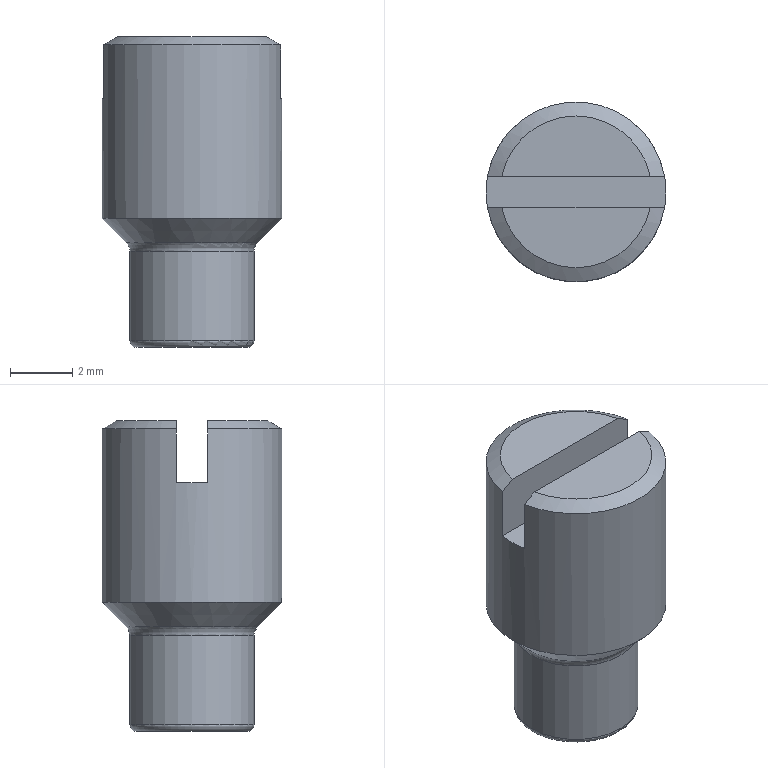Component | NX | SET_SCREW | 1 solid | 13 faces | box 5.8 x 5.8 x 10 mm | volume 200 mm3 | plane 6 | cone 3 | cylinder 2 | torus 2 | commonest cylinder face diameters 5.795 x1 4 x1
STEP:
#1=CARTESIAN_POINT('',(0.,0.,0.));
#2=DIRECTION('',(0.,0.,1.));
#3=DIRECTION('',(1.,0.,0.));
#4=AXIS2_PLACEMENT_3D('',#1,#2,#3);
#5=CARTESIAN_POINT('',(55.394,0.5,23.5));
#6=VERTEX_POINT('',#5);
#7=CARTESIAN_POINT('',(50.606,0.5,23.5));
#8=VERTEX_POINT('',#7);
#9=CARTESIAN_POINT('',(58.795,0.5,23.5));
#10=DIRECTION('',(-1.,0.,0.));
#11=VECTOR('',#10,1.);
#12=LINE('',#9,#11);
#13=CARTESIAN_POINT('',(53.,2.446,23.5));
#14=DIRECTION('',(0.,0.,-1.));
#15=DIRECTION('',(-1.,0.,0.));
#16=AXIS2_PLACEMENT_3D('',#13,#14,#15);
#17=PLANE('',#16);
#18=CARTESIAN_POINT('',(-5.795,-1.946));
#19=DIRECTION('',(1.,0.));
#20=VECTOR('',#19,1.);
#21=LINE('',#18,#20);
#22=(GEOMETRIC_REPRESENTATION_CONTEXT(2)PARAMETRIC_REPRESENTATION_CONTEXT()REPRESENTATION_CONTEXT('',''));
#23=DEFINITIONAL_REPRESENTATION('',(#21),#22);
#24=PCURVE('',#17,#23);
#25=CARTESIAN_POINT('',(58.795,0.5,23.5));
#26=DIRECTION('',(0.,1.,0.));
#27=DIRECTION('',(0.,-0.,1.));
#28=AXIS2_PLACEMENT_3D('',#25,#26,#27);
#29=PLANE('',#28);
#30=CARTESIAN_POINT('',(0.,0.));
#31=DIRECTION('',(0.,-1.));
#32=VECTOR('',#31,1.);
#33=LINE('',#30,#32);
#34=(GEOMETRIC_REPRESENTATION_CONTEXT(2)PARAMETRIC_REPRESENTATION_CONTEXT()REPRESENTATION_CONTEXT('',''));
#35=DEFINITIONAL_REPRESENTATION('',(#33),#34);
#36=PCURVE('',#29,#35);
#37=SURFACE_CURVE('',#12,(#24,#36),.PCURVE_S1.);
#38=EDGE_CURVE('',#6,#8,#37,.T.);
#39=ORIENTED_EDGE('',*,*,#38,.F.);
#40=CARTESIAN_POINT('',(53.,-0.,23.5));
#41=DIRECTION('',(0.,0.,1.));
#42=DIRECTION('',(1.,0.,0.));
#43=AXIS2_PLACEMENT_3D('',#40,#41,#42);
#44=CIRCLE('',#43,2.446);
#45=CARTESIAN_POINT('',(-2.446,-2.446));
#46=CARTESIAN_POINT('',(-2.446,1.79));
#47=CARTESIAN_POINT('',(1.223,-0.3276));
#48=CARTESIAN_POINT('',(4.891,-2.446));
#49=CARTESIAN_POINT('',(1.223,-4.563));
#50=CARTESIAN_POINT('',(-2.446,-6.681));
#51=CARTESIAN_POINT('',(-2.446,-2.446));
#52=(BOUNDED_CURVE()B_SPLINE_CURVE(2,(#45,#46,#47,#48,#49,#50,#51),.UNSPECIFIED.,.T.,.F.)B_SPLINE_CURVE_WITH_KNOTS((1,2,2,2,2,1),(-2.094,0.,2.094,4.189,6.283,8.378),.UNSPECIFIED.)CURVE()GEOMETRIC_REPRESENTATION_ITEM()RATIONAL_B_SPLINE_CURVE((1.,0.5,1.,0.5,1.,0.5,1.))REPRESENTATION_ITEM(''));
#53=(GEOMETRIC_REPRESENTATION_CONTEXT(2)PARAMETRIC_REPRESENTATION_CONTEXT()REPRESENTATION_CONTEXT('',''));
#54=DEFINITIONAL_REPRESENTATION('',(#52),#53);
#55=PCURVE('',#17,#54);
#56=CARTESIAN_POINT('',(53.,-0.,23.239));
#57=DIRECTION('',(0.,0.,-1.));
#58=DIRECTION('',(-1.,0.,0.));
#59=AXIS2_PLACEMENT_3D('',#56,#57,#58);
#60=CONICAL_SURFACE('',#59,2.897,1.047);
#61=CARTESIAN_POINT('',(3.142,-0.261));
#62=DIRECTION('',(-1.,0.));
#63=VECTOR('',#62,1.);
#64=LINE('',#61,#63);
#65=(GEOMETRIC_REPRESENTATION_CONTEXT(2)PARAMETRIC_REPRESENTATION_CONTEXT()REPRESENTATION_CONTEXT('',''));
#66=DEFINITIONAL_REPRESENTATION('',(#64),#65);
#67=PCURVE('',#60,#66);
#68=SURFACE_CURVE('',#44,(#55,#67),.PCURVE_S1.);
#69=EDGE_CURVE('',#6,#8,#68,.T.);
#70=ORIENTED_EDGE('',*,*,#69,.T.);
#71=EDGE_LOOP('',(#39,#70));
#72=FACE_BOUND('',#71,.T.);
#73=ADVANCED_FACE('',(#72),#17,.F.);
#74=CARTESIAN_POINT('',(55.854,0.5,23.239));
#75=VERTEX_POINT('',#74);
#76=CARTESIAN_POINT('',(50.146,0.5,23.239));
#77=VERTEX_POINT('',#76);
#78=CARTESIAN_POINT('',(53.,-0.,23.239));
#79=DIRECTION('',(0.,0.,1.));
#80=DIRECTION('',(1.,0.,0.));
#81=AXIS2_PLACEMENT_3D('',#78,#79,#80);
#82=CIRCLE('',#81,2.897);
#83=CARTESIAN_POINT('',(3.142,-0.));
#84=DIRECTION('',(-1.,0.));
#85=VECTOR('',#84,1.);
#86=LINE('',#83,#85);
#87=(GEOMETRIC_REPRESENTATION_CONTEXT(2)PARAMETRIC_REPRESENTATION_CONTEXT()REPRESENTATION_CONTEXT('',''));
#88=DEFINITIONAL_REPRESENTATION('',(#86),#87);
#89=PCURVE('',#60,#88);
#90=CARTESIAN_POINT('',(53.,-0.,23.5));
#91=DIRECTION('',(0.,0.,1.));
#92=DIRECTION('',(1.,0.,0.));
#93=AXIS2_PLACEMENT_3D('',#90,#91,#92);
#94=CYLINDRICAL_SURFACE('',#93,2.897);
#95=CARTESIAN_POINT('',(0.,-0.261));
#96=DIRECTION('',(1.,0.));
#97=VECTOR('',#96,1.);
#98=LINE('',#95,#97);
#99=(GEOMETRIC_REPRESENTATION_CONTEXT(2)PARAMETRIC_REPRESENTATION_CONTEXT()REPRESENTATION_CONTEXT('',''));
#100=DEFINITIONAL_REPRESENTATION('',(#98),#99);
#101=PCURVE('',#94,#100);
#102=SURFACE_CURVE('',#82,(#89,#101),.PCURVE_S1.);
#103=EDGE_CURVE('',#75,#77,#102,.T.);
#104=ORIENTED_EDGE('',*,*,#103,.T.);
#105=CARTESIAN_POINT('',(50.146,0.5,23.239));
#106=CARTESIAN_POINT('',(50.299,0.5,23.326));
#107=CARTESIAN_POINT('',(50.453,0.5,23.413));
#108=CARTESIAN_POINT('',(50.606,0.5,23.5));
#109=B_SPLINE_CURVE_WITH_KNOTS('',3,(#105,#106,#107,#108),.UNSPECIFIED.,.F.,.F.,(4,4),(0.,1.),.PIECEWISE_BEZIER_KNOTS.);
#110=CARTESIAN_POINT('',(0.1734,-0.));
#111=CARTESIAN_POINT('',(0.2059,-0.261));
#112=B_SPLINE_CURVE_WITH_KNOTS('',1,(#110,#111),.UNSPECIFIED.,.F.,.F.,(2,2),(0.,1.),.PIECEWISE_BEZIER_KNOTS.);
#113=(GEOMETRIC_REPRESENTATION_CONTEXT(2)PARAMETRIC_REPRESENTATION_CONTEXT()REPRESENTATION_CONTEXT('',''));
#114=DEFINITIONAL_REPRESENTATION('',(#112),#113);
#115=PCURVE('',#60,#114);
#116=CARTESIAN_POINT('',(-0.261,-8.649));
#117=CARTESIAN_POINT('',(-0.1738,-8.496));
#118=CARTESIAN_POINT('',(-0.08676,-8.342));
#119=CARTESIAN_POINT('',(0.,-8.189));
#120=B_SPLINE_CURVE_WITH_KNOTS('',3,(#116,#117,#118,#119),.UNSPECIFIED.,.F.,.F.,(4,4),(0.,1.),.PIECEWISE_BEZIER_KNOTS.);
#121=(GEOMETRIC_REPRESENTATION_CONTEXT(2)PARAMETRIC_REPRESENTATION_CONTEXT()REPRESENTATION_CONTEXT('',''));
#122=DEFINITIONAL_REPRESENTATION('',(#120),#121);
#123=PCURVE('',#29,#122);
#124=SURFACE_CURVE('',#109,(#115,#123),.PCURVE_S1.);
#125=EDGE_CURVE('',#77,#8,#124,.T.);
#126=ORIENTED_EDGE('',*,*,#125,.T.);
#127=ORIENTED_EDGE('',*,*,#69,.F.);
#128=CARTESIAN_POINT('',(55.394,0.5,23.5));
#129=CARTESIAN_POINT('',(55.547,0.5,23.413));
#130=CARTESIAN_POINT('',(55.701,0.5,23.326));
#131=CARTESIAN_POINT('',(55.854,0.5,23.239));
#132=B_SPLINE_CURVE_WITH_KNOTS('',3,(#128,#129,#130,#131),.UNSPECIFIED.,.F.,.F.,(4,4),(0.,1.),.PIECEWISE_BEZIER_KNOTS.);
#133=CARTESIAN_POINT('',(2.936,-0.261));
#134=CARTESIAN_POINT('',(2.968,-0.));
#135=B_SPLINE_CURVE_WITH_KNOTS('',1,(#133,#134),.UNSPECIFIED.,.F.,.F.,(2,2),(0.,1.),.PIECEWISE_BEZIER_KNOTS.);
#136=(GEOMETRIC_REPRESENTATION_CONTEXT(2)PARAMETRIC_REPRESENTATION_CONTEXT()REPRESENTATION_CONTEXT('',''));
#137=DEFINITIONAL_REPRESENTATION('',(#135),#136);
#138=PCURVE('',#60,#137);
#139=CARTESIAN_POINT('',(0.,-3.401));
#140=CARTESIAN_POINT('',(-0.08676,-3.248));
#141=CARTESIAN_POINT('',(-0.1738,-3.094));
#142=CARTESIAN_POINT('',(-0.261,-2.941));
#143=B_SPLINE_CURVE_WITH_KNOTS('',3,(#139,#140,#141,#142),.UNSPECIFIED.,.F.,.F.,(4,4),(0.,1.),.PIECEWISE_BEZIER_KNOTS.);
#144=(GEOMETRIC_REPRESENTATION_CONTEXT(2)PARAMETRIC_REPRESENTATION_CONTEXT()REPRESENTATION_CONTEXT('',''));
#145=DEFINITIONAL_REPRESENTATION('',(#143),#144);
#146=PCURVE('',#29,#145);
#147=SURFACE_CURVE('',#132,(#138,#146),.PCURVE_S1.);
#148=EDGE_CURVE('',#6,#75,#147,.T.);
#149=ORIENTED_EDGE('',*,*,#148,.T.);
#150=EDGE_LOOP('',(#104,#126,#127,#149));
#151=FACE_BOUND('',#150,.T.);
#152=ADVANCED_FACE('',(#151),#60,.T.);
#153=CARTESIAN_POINT('',(50.606,-0.5,23.5));
#154=VERTEX_POINT('',#153);
#155=CARTESIAN_POINT('',(55.394,-0.5,23.5));
#156=VERTEX_POINT('',#155);
#157=CARTESIAN_POINT('',(53.,-0.,23.5));
#158=DIRECTION('',(0.,0.,1.));
#159=DIRECTION('',(1.,0.,0.));
#160=AXIS2_PLACEMENT_3D('',#157,#158,#159);
#161=CIRCLE('',#160,2.446);
#162=CARTESIAN_POINT('',(53.,2.446,23.5));
#163=DIRECTION('',(0.,0.,-1.));
#164=DIRECTION('',(-1.,0.,0.));
#165=AXIS2_PLACEMENT_3D('',#162,#163,#164);
#166=PLANE('',#165);
#167=CARTESIAN_POINT('',(-2.446,-2.446));
#168=CARTESIAN_POINT('',(-2.446,1.79));
#169=CARTESIAN_POINT('',(1.223,-0.3276));
#170=CARTESIAN_POINT('',(4.891,-2.446));
#171=CARTESIAN_POINT('',(1.223,-4.563));
#172=CARTESIAN_POINT('',(-2.446,-6.681));
#173=CARTESIAN_POINT('',(-2.446,-2.446));
#174=(BOUNDED_CURVE()B_SPLINE_CURVE(2,(#167,#168,#169,#170,#171,#172,#173),.UNSPECIFIED.,.T.,.F.)B_SPLINE_CURVE_WITH_KNOTS((1,2,2,2,2,1),(-2.094,0.,2.094,4.189,6.283,8.378),.UNSPECIFIED.)CURVE()GEOMETRIC_REPRESENTATION_ITEM()RATIONAL_B_SPLINE_CURVE((1.,0.5,1.,0.5,1.,0.5,1.))REPRESENTATION_ITEM(''));
#175=(GEOMETRIC_REPRESENTATION_CONTEXT(2)PARAMETRIC_REPRESENTATION_CONTEXT()REPRESENTATION_CONTEXT('',''));
#176=DEFINITIONAL_REPRESENTATION('',(#174),#175);
#177=PCURVE('',#166,#176);
#178=CARTESIAN_POINT('',(53.,-0.,23.239));
#179=DIRECTION('',(0.,0.,-1.));
#180=DIRECTION('',(-1.,0.,0.));
#181=AXIS2_PLACEMENT_3D('',#178,#179,#180);
#182=CONICAL_SURFACE('',#181,2.897,1.047);
#183=CARTESIAN_POINT('',(9.425,-0.261));
#184=DIRECTION('',(-1.,0.));
#185=VECTOR('',#184,1.);
#186=LINE('',#183,#185);
#187=(GEOMETRIC_REPRESENTATION_CONTEXT(2)PARAMETRIC_REPRESENTATION_CONTEXT()REPRESENTATION_CONTEXT('',''));
#188=DEFINITIONAL_REPRESENTATION('',(#186),#187);
#189=PCURVE('',#182,#188);
#190=SURFACE_CURVE('',#161,(#177,#189),.PCURVE_S1.);
#191=EDGE_CURVE('',#154,#156,#190,.T.);
#192=ORIENTED_EDGE('',*,*,#191,.T.);
#193=CARTESIAN_POINT('',(58.795,-0.5,23.5));
#194=DIRECTION('',(-1.,0.,0.));
#195=VECTOR('',#194,1.);
#196=LINE('',#193,#195);
#197=CARTESIAN_POINT('',(-5.795,-2.946));
#198=DIRECTION('',(1.,0.));
#199=VECTOR('',#198,1.);
#200=LINE('',#197,#199);
#201=(GEOMETRIC_REPRESENTATION_CONTEXT(2)PARAMETRIC_REPRESENTATION_CONTEXT()REPRESENTATION_CONTEXT('',''));
#202=DEFINITIONAL_REPRESENTATION('',(#200),#201);
#203=PCURVE('',#166,#202);
#204=CARTESIAN_POINT('',(58.795,-0.5,21.5));
#205=DIRECTION('',(0.,-1.,0.));
#206=DIRECTION('',(0.,-0.,-1.));
#207=AXIS2_PLACEMENT_3D('',#204,#205,#206);
#208=PLANE('',#207);
#209=CARTESIAN_POINT('',(-2.,0.));
#210=DIRECTION('',(0.,-1.));
#211=VECTOR('',#210,1.);
#212=LINE('',#209,#211);
#213=(GEOMETRIC_REPRESENTATION_CONTEXT(2)PARAMETRIC_REPRESENTATION_CONTEXT()REPRESENTATION_CONTEXT('',''));
#214=DEFINITIONAL_REPRESENTATION('',(#212),#213);
#215=PCURVE('',#208,#214);
#216=SURFACE_CURVE('',#196,(#203,#215),.PCURVE_S1.);
#217=EDGE_CURVE('',#156,#154,#216,.T.);
#218=ORIENTED_EDGE('',*,*,#217,.T.);
#219=EDGE_LOOP('',(#192,#218));
#220=FACE_BOUND('',#219,.T.);
#221=ADVANCED_FACE('',(#220),#166,.F.);
#222=CARTESIAN_POINT('',(50.146,-0.5,23.239));
#223=VERTEX_POINT('',#222);
#224=CARTESIAN_POINT('',(55.854,-0.5,23.239));
#225=VERTEX_POINT('',#224);
#226=CARTESIAN_POINT('',(53.,-0.,23.239));
#227=DIRECTION('',(0.,0.,1.));
#228=DIRECTION('',(1.,0.,0.));
#229=AXIS2_PLACEMENT_3D('',#226,#227,#228);
#230=CIRCLE('',#229,2.897);
#231=CARTESIAN_POINT('',(9.425,-0.));
#232=DIRECTION('',(-1.,0.));
#233=VECTOR('',#232,1.);
#234=LINE('',#231,#233);
#235=(GEOMETRIC_REPRESENTATION_CONTEXT(2)PARAMETRIC_REPRESENTATION_CONTEXT()REPRESENTATION_CONTEXT('',''));
#236=DEFINITIONAL_REPRESENTATION('',(#234),#235);
#237=PCURVE('',#182,#236);
#238=CARTESIAN_POINT('',(0.,-0.261));
#239=DIRECTION('',(1.,0.));
#240=VECTOR('',#239,1.);
#241=LINE('',#238,#240);
#242=(GEOMETRIC_REPRESENTATION_CONTEXT(2)PARAMETRIC_REPRESENTATION_CONTEXT()REPRESENTATION_CONTEXT('',''));
#243=DEFINITIONAL_REPRESENTATION('',(#241),#242);
#244=PCURVE('',#94,#243);
#245=SURFACE_CURVE('',#230,(#237,#244),.PCURVE_S1.);
#246=EDGE_CURVE('',#223,#225,#245,.T.);
#247=ORIENTED_EDGE('',*,*,#246,.T.);
#248=CARTESIAN_POINT('',(55.854,-0.5,23.239));
#249=CARTESIAN_POINT('',(55.701,-0.5,23.326));
#250=CARTESIAN_POINT('',(55.547,-0.5,23.413));
#251=CARTESIAN_POINT('',(55.394,-0.5,23.5));
#252=B_SPLINE_CURVE_WITH_KNOTS('',3,(#248,#249,#250,#251),.UNSPECIFIED.,.F.,.F.,(4,4),(0.,1.),.PIECEWISE_BEZIER_KNOTS.);
#253=CARTESIAN_POINT('',(3.315,-0.));
#254=CARTESIAN_POINT('',(3.348,-0.261));
#255=B_SPLINE_CURVE_WITH_KNOTS('',1,(#253,#254),.UNSPECIFIED.,.F.,.F.,(2,2),(0.,1.),.PIECEWISE_BEZIER_KNOTS.);
#256=(GEOMETRIC_REPRESENTATION_CONTEXT(2)PARAMETRIC_REPRESENTATION_CONTEXT()REPRESENTATION_CONTEXT('',''));
#257=DEFINITIONAL_REPRESENTATION('',(#255),#256);
#258=PCURVE('',#182,#257);
#259=CARTESIAN_POINT('',(-1.739,-2.941));
#260=CARTESIAN_POINT('',(-1.826,-3.094));
#261=CARTESIAN_POINT('',(-1.913,-3.248));
#262=CARTESIAN_POINT('',(-2.,-3.401));
#263=B_SPLINE_CURVE_WITH_KNOTS('',3,(#259,#260,#261,#262),.UNSPECIFIED.,.F.,.F.,(4,4),(0.,1.),.PIECEWISE_BEZIER_KNOTS.);
#264=(GEOMETRIC_REPRESENTATION_CONTEXT(2)PARAMETRIC_REPRESENTATION_CONTEXT()REPRESENTATION_CONTEXT('',''));
#265=DEFINITIONAL_REPRESENTATION('',(#263),#264);
#266=PCURVE('',#208,#265);
#267=SURFACE_CURVE('',#252,(#258,#266),.PCURVE_S1.);
#268=EDGE_CURVE('',#225,#156,#267,.T.);
#269=ORIENTED_EDGE('',*,*,#268,.T.);
#270=ORIENTED_EDGE('',*,*,#191,.F.);
#271=CARTESIAN_POINT('',(50.606,-0.5,23.5));
#272=CARTESIAN_POINT('',(50.453,-0.5,23.413));
#273=CARTESIAN_POINT('',(50.299,-0.5,23.326));
#274=CARTESIAN_POINT('',(50.146,-0.5,23.239));
#275=B_SPLINE_CURVE_WITH_KNOTS('',3,(#271,#272,#273,#274),.UNSPECIFIED.,.F.,.F.,(4,4),(0.,1.),.PIECEWISE_BEZIER_KNOTS.);
#276=CARTESIAN_POINT('',(6.077,-0.261));
#277=CARTESIAN_POINT('',(6.11,-0.));
#278=B_SPLINE_CURVE_WITH_KNOTS('',1,(#276,#277),.UNSPECIFIED.,.F.,.F.,(2,2),(0.,1.),.PIECEWISE_BEZIER_KNOTS.);
#279=(GEOMETRIC_REPRESENTATION_CONTEXT(2)PARAMETRIC_REPRESENTATION_CONTEXT()REPRESENTATION_CONTEXT('',''));
#280=DEFINITIONAL_REPRESENTATION('',(#278),#279);
#281=PCURVE('',#182,#280);
#282=CARTESIAN_POINT('',(-2.,-8.189));
#283=CARTESIAN_POINT('',(-1.913,-8.342));
#284=CARTESIAN_POINT('',(-1.826,-8.496));
#285=CARTESIAN_POINT('',(-1.739,-8.649));
#286=B_SPLINE_CURVE_WITH_KNOTS('',3,(#282,#283,#284,#285),.UNSPECIFIED.,.F.,.F.,(4,4),(0.,1.),.PIECEWISE_BEZIER_KNOTS.);
#287=(GEOMETRIC_REPRESENTATION_CONTEXT(2)PARAMETRIC_REPRESENTATION_CONTEXT()REPRESENTATION_CONTEXT('',''));
#288=DEFINITIONAL_REPRESENTATION('',(#286),#287);
#289=PCURVE('',#208,#288);
#290=SURFACE_CURVE('',#275,(#281,#289),.PCURVE_S1.);
#291=EDGE_CURVE('',#154,#223,#290,.T.);
#292=ORIENTED_EDGE('',*,*,#291,.T.);
#293=EDGE_LOOP('',(#247,#269,#270,#292));
#294=FACE_BOUND('',#293,.T.);
#295=ADVANCED_FACE('',(#294),#182,.T.);
#296=ORIENTED_EDGE('',*,*,#103,.F.);
#297=CARTESIAN_POINT('',(55.854,0.5,21.5));
#298=VERTEX_POINT('',#297);
#299=CARTESIAN_POINT('',(55.854,0.5,23.5));
#300=DIRECTION('',(0.,0.,-1.));
#301=VECTOR('',#300,1.);
#302=LINE('',#299,#301);
#303=CARTESIAN_POINT('',(0.1734,0.));
#304=DIRECTION('',(0.,-1.));
#305=VECTOR('',#304,1.);
#306=LINE('',#303,#305);
#307=(GEOMETRIC_REPRESENTATION_CONTEXT(2)PARAMETRIC_REPRESENTATION_CONTEXT()REPRESENTATION_CONTEXT('',''));
#308=DEFINITIONAL_REPRESENTATION('',(#306),#307);
#309=PCURVE('',#94,#308);
#310=CARTESIAN_POINT('',(0.,-2.941));
#311=DIRECTION('',(-1.,0.));
#312=VECTOR('',#311,1.);
#313=LINE('',#310,#312);
#314=(GEOMETRIC_REPRESENTATION_CONTEXT(2)PARAMETRIC_REPRESENTATION_CONTEXT()REPRESENTATION_CONTEXT('',''));
#315=DEFINITIONAL_REPRESENTATION('',(#313),#314);
#316=PCURVE('',#29,#315);
#317=SURFACE_CURVE('',#302,(#309,#316),.PCURVE_S1.);
#318=EDGE_CURVE('',#75,#298,#317,.T.);
#319=ORIENTED_EDGE('',*,*,#318,.T.);
#320=CARTESIAN_POINT('',(55.898,-0.,21.5));
#321=VERTEX_POINT('',#320);
#322=CARTESIAN_POINT('',(53.,-0.,21.5));
#323=DIRECTION('',(0.,0.,-1.));
#324=DIRECTION('',(-1.,0.,0.));
#325=AXIS2_PLACEMENT_3D('',#322,#323,#324);
#326=CIRCLE('',#325,2.897);
#327=CARTESIAN_POINT('',(3.142,-2.));
#328=DIRECTION('',(-1.,0.));
#329=VECTOR('',#328,1.);
#330=LINE('',#327,#329);
#331=(GEOMETRIC_REPRESENTATION_CONTEXT(2)PARAMETRIC_REPRESENTATION_CONTEXT()REPRESENTATION_CONTEXT('',''));
#332=DEFINITIONAL_REPRESENTATION('',(#330),#331);
#333=PCURVE('',#94,#332);
#334=CARTESIAN_POINT('',(58.795,-0.,21.5));
#335=DIRECTION('',(0.,0.,-1.));
#336=DIRECTION('',(-1.,0.,0.));
#337=AXIS2_PLACEMENT_3D('',#334,#335,#336);
#338=PLANE('',#337);
#339=CARTESIAN_POINT('',(5.795,0.));
#340=DIRECTION('',(1.,0.));
#341=AXIS2_PLACEMENT_2D('',#339,#340);
#342=CIRCLE('',#341,2.897);
#343=(GEOMETRIC_REPRESENTATION_CONTEXT(2)PARAMETRIC_REPRESENTATION_CONTEXT()REPRESENTATION_CONTEXT('',''));
#344=DEFINITIONAL_REPRESENTATION('',(#342),#343);
#345=PCURVE('',#338,#344);
#346=SURFACE_CURVE('',#326,(#333,#345),.PCURVE_S1.);
#347=EDGE_CURVE('',#298,#321,#346,.T.);
#348=ORIENTED_EDGE('',*,*,#347,.T.);
#349=CARTESIAN_POINT('',(55.898,-0.,17.648));
#350=VERTEX_POINT('',#349);
#351=CARTESIAN_POINT('',(55.898,-0.,17.648));
#352=CARTESIAN_POINT('',(55.898,-0.,21.5));
#353=B_SPLINE_CURVE_WITH_KNOTS('',1,(#351,#352),.UNSPECIFIED.,.F.,.F.,(2,2),(-5.853,-2.),.PIECEWISE_BEZIER_KNOTS.);
#354=CARTESIAN_POINT('',(0.,0.));
#355=DIRECTION('',(0.,1.));
#356=VECTOR('',#355,1.);
#357=LINE('',#354,#356);
#358=(GEOMETRIC_REPRESENTATION_CONTEXT(2)PARAMETRIC_REPRESENTATION_CONTEXT()REPRESENTATION_CONTEXT('',''));
#359=DEFINITIONAL_REPRESENTATION('',(#357),#358);
#360=PCURVE('',#94,#359);
#361=CARTESIAN_POINT('',(6.283,0.));
#362=DIRECTION('',(0.,1.));
#363=VECTOR('',#362,1.);
#364=LINE('',#361,#363);
#365=(GEOMETRIC_REPRESENTATION_CONTEXT(2)PARAMETRIC_REPRESENTATION_CONTEXT()REPRESENTATION_CONTEXT('',''));
#366=DEFINITIONAL_REPRESENTATION('',(#364),#365);
#367=PCURVE('',#94,#366);
#368=SEAM_CURVE('',#353,(#360,#367),.PCURVE_S1.);
#369=EDGE_CURVE('',#350,#321,#368,.T.);
#370=ORIENTED_EDGE('',*,*,#369,.F.);
#371=CARTESIAN_POINT('',(53.,-0.,17.648));
#372=DIRECTION('',(0.,0.,1.));
#373=DIRECTION('',(1.,0.,0.));
#374=AXIS2_PLACEMENT_3D('',#371,#372,#373);
#375=CIRCLE('',#374,2.897);
#376=CARTESIAN_POINT('',(0.,-5.853));
#377=DIRECTION('',(1.,0.));
#378=VECTOR('',#377,1.);
#379=LINE('',#376,#378);
#380=(GEOMETRIC_REPRESENTATION_CONTEXT(2)PARAMETRIC_REPRESENTATION_CONTEXT()REPRESENTATION_CONTEXT('',''));
#381=DEFINITIONAL_REPRESENTATION('',(#379),#380);
#382=PCURVE('',#94,#381);
#383=CARTESIAN_POINT('',(53.,-0.,16.75));
#384=DIRECTION('',(0.,0.,1.));
#385=DIRECTION('',(1.,0.,0.));
#386=AXIS2_PLACEMENT_3D('',#383,#384,#385);
#387=CONICAL_SURFACE('',#386,2.,0.7854);
#388=CARTESIAN_POINT('',(0.,0.8975));
#389=DIRECTION('',(1.,0.));
#390=VECTOR('',#389,1.);
#391=LINE('',#388,#390);
#392=(GEOMETRIC_REPRESENTATION_CONTEXT(2)PARAMETRIC_REPRESENTATION_CONTEXT()REPRESENTATION_CONTEXT('',''));
#393=DEFINITIONAL_REPRESENTATION('',(#391),#392);
#394=PCURVE('',#387,#393);
#395=SURFACE_CURVE('',#375,(#382,#394),.PCURVE_S1.);
#396=EDGE_CURVE('',#350,#350,#395,.T.);
#397=ORIENTED_EDGE('',*,*,#396,.T.);
#398=ORIENTED_EDGE('',*,*,#369,.T.);
#399=CARTESIAN_POINT('',(55.854,-0.5,21.5));
#400=VERTEX_POINT('',#399);
#401=CARTESIAN_POINT('',(53.,-0.,21.5));
#402=DIRECTION('',(0.,0.,-1.));
#403=DIRECTION('',(-1.,0.,0.));
#404=AXIS2_PLACEMENT_3D('',#401,#402,#403);
#405=CIRCLE('',#404,2.897);
#406=CARTESIAN_POINT('',(9.425,-2.));
#407=DIRECTION('',(-1.,0.));
#408=VECTOR('',#407,1.);
#409=LINE('',#406,#408);
#410=(GEOMETRIC_REPRESENTATION_CONTEXT(2)PARAMETRIC_REPRESENTATION_CONTEXT()REPRESENTATION_CONTEXT('',''));
#411=DEFINITIONAL_REPRESENTATION('',(#409),#410);
#412=PCURVE('',#94,#411);
#413=CARTESIAN_POINT('',(5.795,0.));
#414=DIRECTION('',(1.,0.));
#415=AXIS2_PLACEMENT_2D('',#413,#414);
#416=CIRCLE('',#415,2.897);
#417=(GEOMETRIC_REPRESENTATION_CONTEXT(2)PARAMETRIC_REPRESENTATION_CONTEXT()REPRESENTATION_CONTEXT('',''));
#418=DEFINITIONAL_REPRESENTATION('',(#416),#417);
#419=PCURVE('',#338,#418);
#420=SURFACE_CURVE('',#405,(#412,#419),.PCURVE_S1.);
#421=EDGE_CURVE('',#321,#400,#420,.T.);
#422=ORIENTED_EDGE('',*,*,#421,.T.);
#423=CARTESIAN_POINT('',(55.854,-0.5,23.5));
#424=DIRECTION('',(0.,0.,1.));
#425=VECTOR('',#424,1.);
#426=LINE('',#423,#425);
#427=CARTESIAN_POINT('',(6.11,0.));
#428=DIRECTION('',(0.,1.));
#429=VECTOR('',#428,1.);
#430=LINE('',#427,#429);
#431=(GEOMETRIC_REPRESENTATION_CONTEXT(2)PARAMETRIC_REPRESENTATION_CONTEXT()REPRESENTATION_CONTEXT('',''));
#432=DEFINITIONAL_REPRESENTATION('',(#430),#431);
#433=PCURVE('',#94,#432);
#434=CARTESIAN_POINT('',(-2.,-2.941));
#435=DIRECTION('',(-1.,0.));
#436=VECTOR('',#435,1.);
#437=LINE('',#434,#436);
#438=(GEOMETRIC_REPRESENTATION_CONTEXT(2)PARAMETRIC_REPRESENTATION_CONTEXT()REPRESENTATION_CONTEXT('',''));
#439=DEFINITIONAL_REPRESENTATION('',(#437),#438);
#440=PCURVE('',#208,#439);
#441=SURFACE_CURVE('',#426,(#433,#440),.PCURVE_S1.);
#442=EDGE_CURVE('',#400,#225,#441,.T.);
#443=ORIENTED_EDGE('',*,*,#442,.T.);
#444=ORIENTED_EDGE('',*,*,#246,.F.);
#445=CARTESIAN_POINT('',(50.146,-0.5,21.5));
#446=VERTEX_POINT('',#445);
#447=CARTESIAN_POINT('',(50.146,-0.5,23.5));
#448=DIRECTION('',(0.,0.,-1.));
#449=VECTOR('',#448,1.);
#450=LINE('',#447,#449);
#451=CARTESIAN_POINT('',(3.315,0.));
#452=DIRECTION('',(0.,-1.));
#453=VECTOR('',#452,1.);
#454=LINE('',#451,#453);
#455=(GEOMETRIC_REPRESENTATION_CONTEXT(2)PARAMETRIC_REPRESENTATION_CONTEXT()REPRESENTATION_CONTEXT('',''));
#456=DEFINITIONAL_REPRESENTATION('',(#454),#455);
#457=PCURVE('',#94,#456);
#458=CARTESIAN_POINT('',(-2.,-8.649));
#459=DIRECTION('',(1.,0.));
#460=VECTOR('',#459,1.);
#461=LINE('',#458,#460);
#462=(GEOMETRIC_REPRESENTATION_CONTEXT(2)PARAMETRIC_REPRESENTATION_CONTEXT()REPRESENTATION_CONTEXT('',''));
#463=DEFINITIONAL_REPRESENTATION('',(#461),#462);
#464=PCURVE('',#208,#463);
#465=SURFACE_CURVE('',#450,(#457,#464),.PCURVE_S1.);
#466=EDGE_CURVE('',#223,#446,#465,.T.);
#467=ORIENTED_EDGE('',*,*,#466,.T.);
#468=CARTESIAN_POINT('',(50.146,0.5,21.5));
#469=VERTEX_POINT('',#468);
#470=CARTESIAN_POINT('',(53.,-0.,21.5));
#471=DIRECTION('',(0.,0.,-1.));
#472=DIRECTION('',(-1.,0.,0.));
#473=AXIS2_PLACEMENT_3D('',#470,#471,#472);
#474=CIRCLE('',#473,2.897);
#475=CARTESIAN_POINT('',(9.425,-2.));
#476=DIRECTION('',(-1.,0.));
#477=VECTOR('',#476,1.);
#478=LINE('',#475,#477);
#479=(GEOMETRIC_REPRESENTATION_CONTEXT(2)PARAMETRIC_REPRESENTATION_CONTEXT()REPRESENTATION_CONTEXT('',''));
#480=DEFINITIONAL_REPRESENTATION('',(#478),#479);
#481=PCURVE('',#94,#480);
#482=CARTESIAN_POINT('',(5.795,0.));
#483=DIRECTION('',(1.,0.));
#484=AXIS2_PLACEMENT_2D('',#482,#483);
#485=CIRCLE('',#484,2.897);
#486=(GEOMETRIC_REPRESENTATION_CONTEXT(2)PARAMETRIC_REPRESENTATION_CONTEXT()REPRESENTATION_CONTEXT('',''));
#487=DEFINITIONAL_REPRESENTATION('',(#485),#486);
#488=PCURVE('',#338,#487);
#489=SURFACE_CURVE('',#474,(#481,#488),.PCURVE_S1.);
#490=EDGE_CURVE('',#446,#469,#489,.T.);
#491=ORIENTED_EDGE('',*,*,#490,.T.);
#492=CARTESIAN_POINT('',(50.146,0.5,23.5));
#493=DIRECTION('',(0.,0.,1.));
#494=VECTOR('',#493,1.);
#495=LINE('',#492,#494);
#496=CARTESIAN_POINT('',(2.968,0.));
#497=DIRECTION('',(0.,1.));
#498=VECTOR('',#497,1.);
#499=LINE('',#496,#498);
#500=(GEOMETRIC_REPRESENTATION_CONTEXT(2)PARAMETRIC_REPRESENTATION_CONTEXT()REPRESENTATION_CONTEXT('',''));
#501=DEFINITIONAL_REPRESENTATION('',(#499),#500);
#502=PCURVE('',#94,#501);
#503=CARTESIAN_POINT('',(0.,-8.649));
#504=DIRECTION('',(1.,0.));
#505=VECTOR('',#504,1.);
#506=LINE('',#503,#505);
#507=(GEOMETRIC_REPRESENTATION_CONTEXT(2)PARAMETRIC_REPRESENTATION_CONTEXT()REPRESENTATION_CONTEXT('',''));
#508=DEFINITIONAL_REPRESENTATION('',(#506),#507);
#509=PCURVE('',#29,#508);
#510=SURFACE_CURVE('',#495,(#502,#509),.PCURVE_S1.);
#511=EDGE_CURVE('',#469,#77,#510,.T.);
#512=ORIENTED_EDGE('',*,*,#511,.T.);
#513=EDGE_LOOP('',(#296,#319,#348,#370,#397,#398,#422,#443,#444,#467,#491,#512));
#514=FACE_BOUND('',#513,.T.);
#515=ADVANCED_FACE('',(#514),#94,.T.);
#516=CARTESIAN_POINT('',(55.113,-0.,16.863));
#517=VERTEX_POINT('',#516);
#518=CARTESIAN_POINT('',(53.,-0.,16.863));
#519=DIRECTION('',(0.,0.,1.));
#520=DIRECTION('',(1.,0.,0.));
#521=AXIS2_PLACEMENT_3D('',#518,#519,#520);
#522=CIRCLE('',#521,2.113);
#523=CARTESIAN_POINT('',(0.,0.1132));
#524=DIRECTION('',(1.,0.));
#525=VECTOR('',#524,1.);
#526=LINE('',#523,#525);
#527=(GEOMETRIC_REPRESENTATION_CONTEXT(2)PARAMETRIC_REPRESENTATION_CONTEXT()REPRESENTATION_CONTEXT('',''));
#528=DEFINITIONAL_REPRESENTATION('',(#526),#527);
#529=PCURVE('',#387,#528);
#530=CARTESIAN_POINT('',(53.,-0.,16.59));
#531=DIRECTION('',(0.,0.,1.));
#532=DIRECTION('',(1.,0.,0.));
#533=AXIS2_PLACEMENT_3D('',#530,#531,#532);
#534=TOROIDAL_SURFACE('',#533,2.386,0.3863);
#535=CARTESIAN_POINT('',(0.,8.639));
#536=DIRECTION('',(1.,0.));
#537=VECTOR('',#536,1.);
#538=LINE('',#535,#537);
#539=(GEOMETRIC_REPRESENTATION_CONTEXT(2)PARAMETRIC_REPRESENTATION_CONTEXT()REPRESENTATION_CONTEXT('',''));
#540=DEFINITIONAL_REPRESENTATION('',(#538),#539);
#541=PCURVE('',#534,#540);
#542=SURFACE_CURVE('',#522,(#529,#541),.PCURVE_S1.);
#543=EDGE_CURVE('',#517,#517,#542,.T.);
#544=ORIENTED_EDGE('',*,*,#543,.T.);
#545=CARTESIAN_POINT('',(55.113,-0.,16.863));
#546=CARTESIAN_POINT('',(55.897,-0.,17.648));
#547=B_SPLINE_CURVE_WITH_KNOTS('',1,(#545,#546),.UNSPECIFIED.,.F.,.F.,(2,2),(0.16,1.269),.PIECEWISE_BEZIER_KNOTS.);
#548=CARTESIAN_POINT('',(6.283,0.));
#549=DIRECTION('',(0.,1.));
#550=VECTOR('',#549,1.);
#551=LINE('',#548,#550);
#552=(GEOMETRIC_REPRESENTATION_CONTEXT(2)PARAMETRIC_REPRESENTATION_CONTEXT()REPRESENTATION_CONTEXT('',''));
#553=DEFINITIONAL_REPRESENTATION('',(#551),#552);
#554=PCURVE('',#387,#553);
#555=CARTESIAN_POINT('',(0.,0.));
#556=DIRECTION('',(0.,1.));
#557=VECTOR('',#556,1.);
#558=LINE('',#555,#557);
#559=(GEOMETRIC_REPRESENTATION_CONTEXT(2)PARAMETRIC_REPRESENTATION_CONTEXT()REPRESENTATION_CONTEXT('',''));
#560=DEFINITIONAL_REPRESENTATION('',(#558),#559);
#561=PCURVE('',#387,#560);
#562=SEAM_CURVE('',#547,(#554,#561),.PCURVE_S1.);
#563=EDGE_CURVE('',#517,#350,#562,.T.);
#564=ORIENTED_EDGE('',*,*,#563,.T.);
#565=ORIENTED_EDGE('',*,*,#396,.F.);
#566=ORIENTED_EDGE('',*,*,#563,.F.);
#567=EDGE_LOOP('',(#544,#564,#565,#566));
#568=FACE_BOUND('',#567,.T.);
#569=ADVANCED_FACE('',(#568),#387,.T.);
#570=CARTESIAN_POINT('',(55.,-0.,16.59));
#571=VERTEX_POINT('',#570);
#572=CARTESIAN_POINT('',(53.,-0.,16.59));
#573=DIRECTION('',(0.,0.,-1.));
#574=DIRECTION('',(1.,0.,0.));
#575=AXIS2_PLACEMENT_3D('',#572,#573,#574);
#576=CIRCLE('',#575,2.);
#577=CARTESIAN_POINT('',(53.,-0.,23.5));
#578=DIRECTION('',(0.,0.,1.));
#579=DIRECTION('',(1.,0.,0.));
#580=AXIS2_PLACEMENT_3D('',#577,#578,#579);
#581=CYLINDRICAL_SURFACE('',#580,2.);
#582=CARTESIAN_POINT('',(6.283,-6.91));
#583=DIRECTION('',(-1.,0.));
#584=VECTOR('',#583,1.);
#585=LINE('',#582,#584);
#586=(GEOMETRIC_REPRESENTATION_CONTEXT(2)PARAMETRIC_REPRESENTATION_CONTEXT()REPRESENTATION_CONTEXT('',''));
#587=DEFINITIONAL_REPRESENTATION('',(#585),#586);
#588=PCURVE('',#581,#587);
#589=CARTESIAN_POINT('',(6.283,9.425));
#590=DIRECTION('',(-1.,0.));
#591=VECTOR('',#590,1.);
#592=LINE('',#589,#591);
#593=(GEOMETRIC_REPRESENTATION_CONTEXT(2)PARAMETRIC_REPRESENTATION_CONTEXT()REPRESENTATION_CONTEXT('',''));
#594=DEFINITIONAL_REPRESENTATION('',(#592),#593);
#595=PCURVE('',#534,#594);
#596=SURFACE_CURVE('',#576,(#588,#595),.PCURVE_S1.);
#597=EDGE_CURVE('',#571,#571,#596,.T.);
#598=ORIENTED_EDGE('',*,*,#597,.T.);
#599=CARTESIAN_POINT('',(55.,-0.,13.7));
#600=VERTEX_POINT('',#599);
#601=CARTESIAN_POINT('',(55.,-0.,13.7));
#602=CARTESIAN_POINT('',(55.,-0.,16.59));
#603=B_SPLINE_CURVE_WITH_KNOTS('',1,(#601,#602),.UNSPECIFIED.,.F.,.F.,(2,2),(-9.8,-6.91),.PIECEWISE_BEZIER_KNOTS.);
#604=CARTESIAN_POINT('',(0.,0.));
#605=DIRECTION('',(0.,1.));
#606=VECTOR('',#605,1.);
#607=LINE('',#604,#606);
#608=(GEOMETRIC_REPRESENTATION_CONTEXT(2)PARAMETRIC_REPRESENTATION_CONTEXT()REPRESENTATION_CONTEXT('',''));
#609=DEFINITIONAL_REPRESENTATION('',(#607),#608);
#610=PCURVE('',#581,#609);
#611=CARTESIAN_POINT('',(6.283,0.));
#612=DIRECTION('',(0.,1.));
#613=VECTOR('',#612,1.);
#614=LINE('',#611,#613);
#615=(GEOMETRIC_REPRESENTATION_CONTEXT(2)PARAMETRIC_REPRESENTATION_CONTEXT()REPRESENTATION_CONTEXT('',''));
#616=DEFINITIONAL_REPRESENTATION('',(#614),#615);
#617=PCURVE('',#581,#616);
#618=SEAM_CURVE('',#603,(#610,#617),.PCURVE_S1.);
#619=EDGE_CURVE('',#600,#571,#618,.T.);
#620=ORIENTED_EDGE('',*,*,#619,.F.);
#621=CARTESIAN_POINT('',(53.,-0.,13.7));
#622=DIRECTION('',(0.,0.,1.));
#623=DIRECTION('',(1.,0.,0.));
#624=AXIS2_PLACEMENT_3D('',#621,#622,#623);
#625=CIRCLE('',#624,2.);
#626=CARTESIAN_POINT('',(0.,-9.8));
#627=DIRECTION('',(1.,0.));
#628=VECTOR('',#627,1.);
#629=LINE('',#626,#628);
#630=(GEOMETRIC_REPRESENTATION_CONTEXT(2)PARAMETRIC_REPRESENTATION_CONTEXT()REPRESENTATION_CONTEXT('',''));
#631=DEFINITIONAL_REPRESENTATION('',(#629),#630);
#632=PCURVE('',#581,#631);
#633=CARTESIAN_POINT('',(53.,-0.,13.7));
#634=DIRECTION('',(0.,0.,1.));
#635=DIRECTION('',(1.,0.,0.));
#636=AXIS2_PLACEMENT_3D('',#633,#634,#635);
#637=TOROIDAL_SURFACE('',#636,1.8,0.2);
#638=CARTESIAN_POINT('',(0.,6.283));
#639=DIRECTION('',(1.,0.));
#640=VECTOR('',#639,1.);
#641=LINE('',#638,#640);
#642=(GEOMETRIC_REPRESENTATION_CONTEXT(2)PARAMETRIC_REPRESENTATION_CONTEXT()REPRESENTATION_CONTEXT('',''));
#643=DEFINITIONAL_REPRESENTATION('',(#641),#642);
#644=PCURVE('',#637,#643);
#645=SURFACE_CURVE('',#625,(#632,#644),.PCURVE_S1.);
#646=EDGE_CURVE('',#600,#600,#645,.T.);
#647=ORIENTED_EDGE('',*,*,#646,.T.);
#648=ORIENTED_EDGE('',*,*,#619,.T.);
#649=EDGE_LOOP('',(#598,#620,#647,#648));
#650=FACE_BOUND('',#649,.T.);
#651=ADVANCED_FACE('',(#650),#581,.T.);
#652=CARTESIAN_POINT('',(54.8,-0.,13.5));
#653=VERTEX_POINT('',#652);
#654=CARTESIAN_POINT('',(53.,-0.,13.5));
#655=DIRECTION('',(0.,0.,-1.));
#656=DIRECTION('',(1.,0.,0.));
#657=AXIS2_PLACEMENT_3D('',#654,#655,#656);
#658=CIRCLE('',#657,1.8);
#659=CARTESIAN_POINT('',(53.,-0.,13.5));
#660=DIRECTION('',(0.,0.,1.));
#661=DIRECTION('',(1.,0.,0.));
#662=AXIS2_PLACEMENT_3D('',#659,#660,#661);
#663=PLANE('',#662);
#664=CARTESIAN_POINT('',(1.8,0.));
#665=CARTESIAN_POINT('',(1.8,-3.118));
#666=CARTESIAN_POINT('',(-0.9,-1.559));
#667=CARTESIAN_POINT('',(-3.6,-0.));
#668=CARTESIAN_POINT('',(-0.9,1.559));
#669=CARTESIAN_POINT('',(1.8,3.118));
#670=CARTESIAN_POINT('',(1.8,0.));
#671=(BOUNDED_CURVE()B_SPLINE_CURVE(2,(#664,#665,#666,#667,#668,#669,#670),.UNSPECIFIED.,.T.,.F.)B_SPLINE_CURVE_WITH_KNOTS((1,2,2,2,2,1),(-2.094,0.,2.094,4.189,6.283,8.378),.UNSPECIFIED.)CURVE()GEOMETRIC_REPRESENTATION_ITEM()RATIONAL_B_SPLINE_CURVE((1.,0.5,1.,0.5,1.,0.5,1.))REPRESENTATION_ITEM(''));
#672=(GEOMETRIC_REPRESENTATION_CONTEXT(2)PARAMETRIC_REPRESENTATION_CONTEXT()REPRESENTATION_CONTEXT('',''));
#673=DEFINITIONAL_REPRESENTATION('',(#671),#672);
#674=PCURVE('',#663,#673);
#675=CARTESIAN_POINT('',(6.283,4.712));
#676=DIRECTION('',(-1.,0.));
#677=VECTOR('',#676,1.);
#678=LINE('',#675,#677);
#679=(GEOMETRIC_REPRESENTATION_CONTEXT(2)PARAMETRIC_REPRESENTATION_CONTEXT()REPRESENTATION_CONTEXT('',''));
#680=DEFINITIONAL_REPRESENTATION('',(#678),#679);
#681=PCURVE('',#637,#680);
#682=SURFACE_CURVE('',#658,(#674,#681),.PCURVE_S1.);
#683=EDGE_CURVE('',#653,#653,#682,.T.);
#684=ORIENTED_EDGE('',*,*,#683,.T.);
#685=EDGE_LOOP('',(#684));
#686=FACE_BOUND('',#685,.T.);
#687=ADVANCED_FACE('',(#686),#663,.F.);
#688=ORIENTED_EDGE('',*,*,#511,.F.);
#689=CARTESIAN_POINT('',(58.795,0.5,21.5));
#690=DIRECTION('',(-1.,0.,0.));
#691=VECTOR('',#690,1.);
#692=LINE('',#689,#691);
#693=CARTESIAN_POINT('',(-2.,0.));
#694=DIRECTION('',(0.,-1.));
#695=VECTOR('',#694,1.);
#696=LINE('',#693,#695);
#697=(GEOMETRIC_REPRESENTATION_CONTEXT(2)PARAMETRIC_REPRESENTATION_CONTEXT()REPRESENTATION_CONTEXT('',''));
#698=DEFINITIONAL_REPRESENTATION('',(#696),#697);
#699=PCURVE('',#29,#698);
#700=CARTESIAN_POINT('',(0.,0.5));
#701=DIRECTION('',(1.,0.));
#702=VECTOR('',#701,1.);
#703=LINE('',#700,#702);
#704=(GEOMETRIC_REPRESENTATION_CONTEXT(2)PARAMETRIC_REPRESENTATION_CONTEXT()REPRESENTATION_CONTEXT('',''));
#705=DEFINITIONAL_REPRESENTATION('',(#703),#704);
#706=PCURVE('',#338,#705);
#707=SURFACE_CURVE('',#692,(#699,#706),.PCURVE_S1.);
#708=EDGE_CURVE('',#298,#469,#707,.T.);
#709=ORIENTED_EDGE('',*,*,#708,.F.);
#710=ORIENTED_EDGE('',*,*,#318,.F.);
#711=ORIENTED_EDGE('',*,*,#148,.F.);
#712=ORIENTED_EDGE('',*,*,#38,.T.);
#713=ORIENTED_EDGE('',*,*,#125,.F.);
#714=EDGE_LOOP('',(#688,#709,#710,#711,#712,#713));
#715=FACE_BOUND('',#714,.T.);
#716=ADVANCED_FACE('',(#715),#29,.F.);
#717=ORIENTED_EDGE('',*,*,#421,.T.);
#718=CARTESIAN_POINT('',(58.795,-0.5,21.5));
#719=DIRECTION('',(-1.,0.,0.));
#720=VECTOR('',#719,1.);
#721=LINE('',#718,#720);
#722=CARTESIAN_POINT('',(0.,-0.5));
#723=DIRECTION('',(1.,0.));
#724=VECTOR('',#723,1.);
#725=LINE('',#722,#724);
#726=(GEOMETRIC_REPRESENTATION_CONTEXT(2)PARAMETRIC_REPRESENTATION_CONTEXT()REPRESENTATION_CONTEXT('',''));
#727=DEFINITIONAL_REPRESENTATION('',(#725),#726);
#728=PCURVE('',#338,#727);
#729=CARTESIAN_POINT('',(0.,0.));
#730=DIRECTION('',(0.,-1.));
#731=VECTOR('',#730,1.);
#732=LINE('',#729,#731);
#733=(GEOMETRIC_REPRESENTATION_CONTEXT(2)PARAMETRIC_REPRESENTATION_CONTEXT()REPRESENTATION_CONTEXT('',''));
#734=DEFINITIONAL_REPRESENTATION('',(#732),#733);
#735=PCURVE('',#208,#734);
#736=SURFACE_CURVE('',#721,(#728,#735),.PCURVE_S1.);
#737=EDGE_CURVE('',#400,#446,#736,.T.);
#738=ORIENTED_EDGE('',*,*,#737,.T.);
#739=ORIENTED_EDGE('',*,*,#490,.T.);
#740=ORIENTED_EDGE('',*,*,#708,.F.);
#741=ORIENTED_EDGE('',*,*,#347,.T.);
#742=EDGE_LOOP('',(#717,#738,#739,#740,#741));
#743=FACE_BOUND('',#742,.F.);
#744=ADVANCED_FACE('',(#743),#338,.F.);
#745=ORIENTED_EDGE('',*,*,#442,.F.);
#746=ORIENTED_EDGE('',*,*,#737,.T.);
#747=ORIENTED_EDGE('',*,*,#466,.F.);
#748=ORIENTED_EDGE('',*,*,#291,.F.);
#749=ORIENTED_EDGE('',*,*,#217,.F.);
#750=ORIENTED_EDGE('',*,*,#268,.F.);
#751=EDGE_LOOP('',(#745,#746,#747,#748,#749,#750));
#752=FACE_BOUND('',#751,.T.);
#753=ADVANCED_FACE('',(#752),#208,.F.);
#754=ORIENTED_EDGE('',*,*,#683,.F.);
#755=CARTESIAN_POINT('',(54.8,-0.,13.5));
#756=CARTESIAN_POINT('',(54.853,-0.,13.5));
#757=CARTESIAN_POINT('',(54.906,-0.,13.517));
#758=CARTESIAN_POINT('',(54.95,-0.,13.55));
#759=CARTESIAN_POINT('',(54.983,-0.,13.594));
#760=CARTESIAN_POINT('',(55.,-0.,13.647));
#761=CARTESIAN_POINT('',(55.,-0.,13.7));
#762=(BOUNDED_CURVE()B_SPLINE_CURVE(6,(#755,#756,#757,#758,#759,#760,#761),.UNSPECIFIED.,.F.,.F.)B_SPLINE_CURVE_WITH_KNOTS((7,7),(4.712,6.283),.PIECEWISE_BEZIER_KNOTS.)CURVE()GEOMETRIC_REPRESENTATION_ITEM()RATIONAL_B_SPLINE_CURVE((1.031,1.01,0.9979,0.994,0.9979,1.01,1.031))REPRESENTATION_ITEM(''));
#763=CARTESIAN_POINT('',(6.283,0.));
#764=DIRECTION('',(0.,1.));
#765=VECTOR('',#764,1.);
#766=LINE('',#763,#765);
#767=(GEOMETRIC_REPRESENTATION_CONTEXT(2)PARAMETRIC_REPRESENTATION_CONTEXT()REPRESENTATION_CONTEXT('',''));
#768=DEFINITIONAL_REPRESENTATION('',(#766),#767);
#769=PCURVE('',#637,#768);
#770=CARTESIAN_POINT('',(0.,0.));
#771=DIRECTION('',(0.,1.));
#772=VECTOR('',#771,1.);
#773=LINE('',#770,#772);
#774=(GEOMETRIC_REPRESENTATION_CONTEXT(2)PARAMETRIC_REPRESENTATION_CONTEXT()REPRESENTATION_CONTEXT('',''));
#775=DEFINITIONAL_REPRESENTATION('',(#773),#774);
#776=PCURVE('',#637,#775);
#777=SEAM_CURVE('',#762,(#769,#776),.PCURVE_S1.);
#778=EDGE_CURVE('',#653,#600,#777,.T.);
#779=ORIENTED_EDGE('',*,*,#778,.T.);
#780=ORIENTED_EDGE('',*,*,#646,.F.);
#781=ORIENTED_EDGE('',*,*,#778,.F.);
#782=EDGE_LOOP('',(#754,#779,#780,#781));
#783=FACE_BOUND('',#782,.T.);
#784=ADVANCED_FACE('',(#783),#637,.T.);
#785=ORIENTED_EDGE('',*,*,#597,.T.);
#786=CARTESIAN_POINT('',(55.113,-0.,16.863));
#787=CARTESIAN_POINT('',(55.077,-0.,16.827));
#788=CARTESIAN_POINT('',(55.047,-0.,16.786));
#789=CARTESIAN_POINT('',(55.024,-0.,16.74));
#790=CARTESIAN_POINT('',(55.008,-0.,16.691));
#791=CARTESIAN_POINT('',(55.,-0.,16.641));
#792=CARTESIAN_POINT('',(55.,-0.,16.59));
#793=(BOUNDED_CURVE()B_SPLINE_CURVE(6,(#786,#787,#788,#789,#790,#791,#792),.UNSPECIFIED.,.F.,.F.)B_SPLINE_CURVE_WITH_KNOTS((7,7),(2.356,3.142),.PIECEWISE_BEZIER_KNOTS.)CURVE()GEOMETRIC_REPRESENTATION_ITEM()RATIONAL_B_SPLINE_CURVE((1.008,1.003,0.9995,0.9985,0.9995,1.003,1.008))REPRESENTATION_ITEM(''));
#794=CARTESIAN_POINT('',(0.,6.283));
#795=DIRECTION('',(0.,1.));
#796=VECTOR('',#795,1.);
#797=LINE('',#794,#796);
#798=(GEOMETRIC_REPRESENTATION_CONTEXT(2)PARAMETRIC_REPRESENTATION_CONTEXT()REPRESENTATION_CONTEXT('',''));
#799=DEFINITIONAL_REPRESENTATION('',(#797),#798);
#800=PCURVE('',#534,#799);
#801=CARTESIAN_POINT('',(6.283,6.283));
#802=DIRECTION('',(0.,1.));
#803=VECTOR('',#802,1.);
#804=LINE('',#801,#803);
#805=(GEOMETRIC_REPRESENTATION_CONTEXT(2)PARAMETRIC_REPRESENTATION_CONTEXT()REPRESENTATION_CONTEXT('',''));
#806=DEFINITIONAL_REPRESENTATION('',(#804),#805);
#807=PCURVE('',#534,#806);
#808=SEAM_CURVE('',#793,(#800,#807),.PCURVE_S1.);
#809=EDGE_CURVE('',#517,#571,#808,.T.);
#810=ORIENTED_EDGE('',*,*,#809,.F.);
#811=ORIENTED_EDGE('',*,*,#543,.T.);
#812=ORIENTED_EDGE('',*,*,#809,.T.);
#813=EDGE_LOOP('',(#785,#810,#811,#812));
#814=FACE_BOUND('',#813,.F.);
#815=ADVANCED_FACE('',(#814),#534,.F.);
#816=CLOSED_SHELL('',(#73,#152,#221,#295,#515,#569,#651,#687,#716,#744,#753,#784,#815));
#817=MANIFOLD_SOLID_BREP('',#816);
#818=(LENGTH_UNIT()NAMED_UNIT(*)SI_UNIT(.MILLI.,.METRE.));
#819=UNCERTAINTY_MEASURE_WITH_UNIT(LENGTH_MEASURE(0.001),#818,'','');
#820=(NAMED_UNIT(*)PLANE_ANGLE_UNIT()SI_UNIT($,.RADIAN.));
#821=(NAMED_UNIT(*)SI_UNIT($,.STERADIAN.)SOLID_ANGLE_UNIT());
#822=(GEOMETRIC_REPRESENTATION_CONTEXT(3)GLOBAL_UNCERTAINTY_ASSIGNED_CONTEXT((#819))GLOBAL_UNIT_ASSIGNED_CONTEXT((#818,#820,#821))REPRESENTATION_CONTEXT('',''));
#823=ADVANCED_BREP_SHAPE_REPRESENTATION('',(#4,#817),#822);